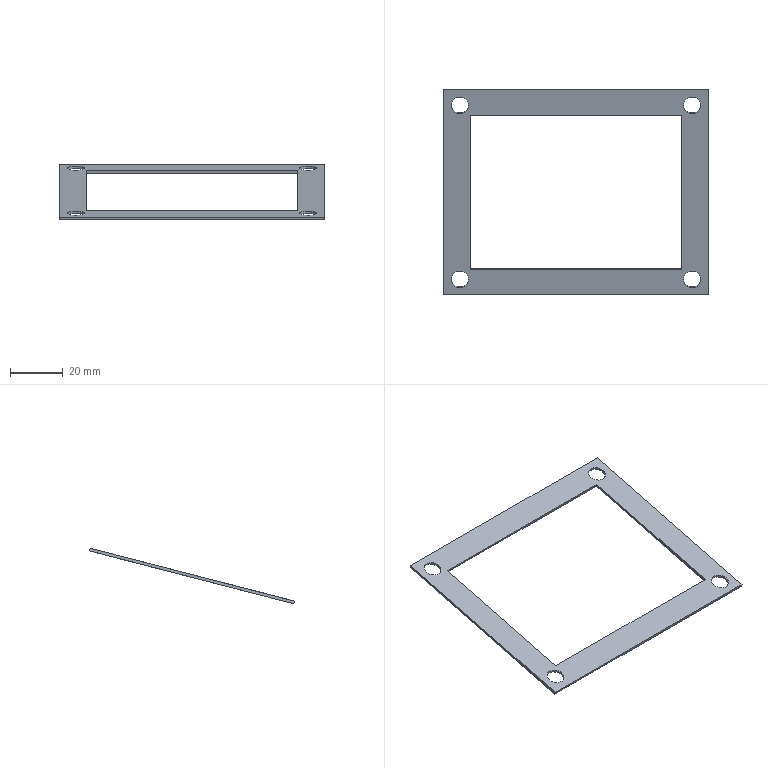Component | NX | DIANPIAN | 1 solid | 14 faces | box 100 x 77.71 x 20.97 mm | volume 3067 mm3 | plane 10 | cylinder 4 | commonest cylinder face diameters 6.5 x4
STEP:
#1=CARTESIAN_POINT('',(0.,0.,0.));
#2=DIRECTION('',(0.,0.,1.));
#3=DIRECTION('',(1.,0.,0.));
#4=AXIS2_PLACEMENT_3D('',#1,#2,#3);
#5=CARTESIAN_POINT('',(-40.,65.493,-7.056));
#6=VERTEX_POINT('',#5);
#7=CARTESIAN_POINT('',(-40.,123.588,7.944));
#8=VERTEX_POINT('',#7);
#9=CARTESIAN_POINT('',(-40.,65.493,-7.056));
#10=DIRECTION('',(0.,0.9682,0.25));
#11=VECTOR('',#10,1.);
#12=LINE('',#9,#11);
#13=CARTESIAN_POINT('',(-40.,65.243,-6.088));
#14=DIRECTION('',(-1.,0.,0.));
#15=DIRECTION('',(0.,-0.25,0.9682));
#16=AXIS2_PLACEMENT_3D('',#13,#14,#15);
#17=PLANE('',#16);
#18=CARTESIAN_POINT('',(-1.,0.));
#19=DIRECTION('',(0.,1.));
#20=VECTOR('',#19,1.);
#21=LINE('',#18,#20);
#22=(GEOMETRIC_REPRESENTATION_CONTEXT(2)PARAMETRIC_REPRESENTATION_CONTEXT()REPRESENTATION_CONTEXT('',''));
#23=DEFINITIONAL_REPRESENTATION('',(#21),#22);
#24=PCURVE('',#17,#23);
#25=CARTESIAN_POINT('',(-44.,61.62,-8.056));
#26=DIRECTION('',(0.,0.25,-0.9682));
#27=DIRECTION('',(-1.,0.,0.));
#28=AXIS2_PLACEMENT_3D('',#25,#26,#27);
#29=PLANE('',#28);
#30=CARTESIAN_POINT('',(-4.,4.));
#31=DIRECTION('',(0.,1.));
#32=VECTOR('',#31,1.);
#33=LINE('',#30,#32);
#34=(GEOMETRIC_REPRESENTATION_CONTEXT(2)PARAMETRIC_REPRESENTATION_CONTEXT()REPRESENTATION_CONTEXT('',''));
#35=DEFINITIONAL_REPRESENTATION('',(#33),#34);
#36=PCURVE('',#29,#35);
#37=SURFACE_CURVE('',#12,(#24,#36),.PCURVE_S1.);
#38=EDGE_CURVE('',#6,#8,#37,.T.);
#39=ORIENTED_EDGE('',*,*,#38,.T.);
#40=CARTESIAN_POINT('',(-40.,123.338,8.912));
#41=VERTEX_POINT('',#40);
#42=CARTESIAN_POINT('',(-40.,123.338,8.912));
#43=DIRECTION('',(0.,0.25,-0.9682));
#44=VECTOR('',#43,1.);
#45=LINE('',#42,#44);
#46=CARTESIAN_POINT('',(0.,60.));
#47=DIRECTION('',(-1.,0.));
#48=VECTOR('',#47,1.);
#49=LINE('',#46,#48);
#50=(GEOMETRIC_REPRESENTATION_CONTEXT(2)PARAMETRIC_REPRESENTATION_CONTEXT()REPRESENTATION_CONTEXT('',''));
#51=DEFINITIONAL_REPRESENTATION('',(#49),#50);
#52=PCURVE('',#17,#51);
#53=CARTESIAN_POINT('',(-40.,123.338,8.912));
#54=DIRECTION('',(0.,0.9682,0.25));
#55=DIRECTION('',(0.,-0.25,0.9682));
#56=AXIS2_PLACEMENT_3D('',#53,#54,#55);
#57=PLANE('',#56);
#58=CARTESIAN_POINT('',(0.,0.));
#59=DIRECTION('',(-1.,0.));
#60=VECTOR('',#59,1.);
#61=LINE('',#58,#60);
#62=(GEOMETRIC_REPRESENTATION_CONTEXT(2)PARAMETRIC_REPRESENTATION_CONTEXT()REPRESENTATION_CONTEXT('',''));
#63=DEFINITIONAL_REPRESENTATION('',(#61),#62);
#64=PCURVE('',#57,#63);
#65=SURFACE_CURVE('',#45,(#52,#64),.PCURVE_S1.);
#66=EDGE_CURVE('',#41,#8,#65,.T.);
#67=ORIENTED_EDGE('',*,*,#66,.F.);
#68=CARTESIAN_POINT('',(-40.,65.243,-6.088));
#69=VERTEX_POINT('',#68);
#70=CARTESIAN_POINT('',(-40.,65.243,-6.088));
#71=DIRECTION('',(0.,0.9682,0.25));
#72=VECTOR('',#71,1.);
#73=LINE('',#70,#72);
#74=CARTESIAN_POINT('',(0.,0.));
#75=DIRECTION('',(0.,1.));
#76=VECTOR('',#75,1.);
#77=LINE('',#74,#76);
#78=(GEOMETRIC_REPRESENTATION_CONTEXT(2)PARAMETRIC_REPRESENTATION_CONTEXT()REPRESENTATION_CONTEXT('',''));
#79=DEFINITIONAL_REPRESENTATION('',(#77),#78);
#80=PCURVE('',#17,#79);
#81=CARTESIAN_POINT('',(-44.,61.37,-7.088));
#82=DIRECTION('',(0.,0.25,-0.9682));
#83=DIRECTION('',(-1.,0.,0.));
#84=AXIS2_PLACEMENT_3D('',#81,#82,#83);
#85=PLANE('',#84);
#86=CARTESIAN_POINT('',(-4.,4.));
#87=DIRECTION('',(0.,1.));
#88=VECTOR('',#87,1.);
#89=LINE('',#86,#88);
#90=(GEOMETRIC_REPRESENTATION_CONTEXT(2)PARAMETRIC_REPRESENTATION_CONTEXT()REPRESENTATION_CONTEXT('',''));
#91=DEFINITIONAL_REPRESENTATION('',(#89),#90);
#92=PCURVE('',#85,#91);
#93=SURFACE_CURVE('',#73,(#80,#92),.PCURVE_S1.);
#94=EDGE_CURVE('',#69,#41,#93,.T.);
#95=ORIENTED_EDGE('',*,*,#94,.F.);
#96=CARTESIAN_POINT('',(-40.,65.243,-6.088));
#97=DIRECTION('',(0.,0.25,-0.9682));
#98=VECTOR('',#97,1.);
#99=LINE('',#96,#98);
#100=CARTESIAN_POINT('',(0.,0.));
#101=DIRECTION('',(-1.,0.));
#102=VECTOR('',#101,1.);
#103=LINE('',#100,#102);
#104=(GEOMETRIC_REPRESENTATION_CONTEXT(2)PARAMETRIC_REPRESENTATION_CONTEXT()REPRESENTATION_CONTEXT('',''));
#105=DEFINITIONAL_REPRESENTATION('',(#103),#104);
#106=PCURVE('',#17,#105);
#107=CARTESIAN_POINT('',(40.,65.243,-6.088));
#108=DIRECTION('',(0.,-0.9682,-0.25));
#109=DIRECTION('',(0.,0.25,-0.9682));
#110=AXIS2_PLACEMENT_3D('',#107,#108,#109);
#111=PLANE('',#110);
#112=CARTESIAN_POINT('',(0.,-80.));
#113=DIRECTION('',(1.,0.));
#114=VECTOR('',#113,1.);
#115=LINE('',#112,#114);
#116=(GEOMETRIC_REPRESENTATION_CONTEXT(2)PARAMETRIC_REPRESENTATION_CONTEXT()REPRESENTATION_CONTEXT('',''));
#117=DEFINITIONAL_REPRESENTATION('',(#115),#116);
#118=PCURVE('',#111,#117);
#119=SURFACE_CURVE('',#99,(#106,#118),.PCURVE_S1.);
#120=EDGE_CURVE('',#69,#6,#119,.T.);
#121=ORIENTED_EDGE('',*,*,#120,.T.);
#122=EDGE_LOOP('',(#39,#67,#95,#121));
#123=FACE_BOUND('',#122,.T.);
#124=ADVANCED_FACE('',(#123),#17,.F.);
#125=CARTESIAN_POINT('',(40.,123.588,7.944));
#126=VERTEX_POINT('',#125);
#127=CARTESIAN_POINT('',(-40.,123.588,7.944));
#128=DIRECTION('',(1.,0.,0.));
#129=VECTOR('',#128,1.);
#130=LINE('',#127,#129);
#131=CARTESIAN_POINT('',(-1.,0.));
#132=DIRECTION('',(0.,1.));
#133=VECTOR('',#132,1.);
#134=LINE('',#131,#133);
#135=(GEOMETRIC_REPRESENTATION_CONTEXT(2)PARAMETRIC_REPRESENTATION_CONTEXT()REPRESENTATION_CONTEXT('',''));
#136=DEFINITIONAL_REPRESENTATION('',(#134),#135);
#137=PCURVE('',#57,#136);
#138=CARTESIAN_POINT('',(-4.,64.));
#139=DIRECTION('',(-1.,0.));
#140=VECTOR('',#139,1.);
#141=LINE('',#138,#140);
#142=(GEOMETRIC_REPRESENTATION_CONTEXT(2)PARAMETRIC_REPRESENTATION_CONTEXT()REPRESENTATION_CONTEXT('',''));
#143=DEFINITIONAL_REPRESENTATION('',(#141),#142);
#144=PCURVE('',#29,#143);
#145=SURFACE_CURVE('',#130,(#137,#144),.PCURVE_S1.);
#146=EDGE_CURVE('',#8,#126,#145,.T.);
#147=ORIENTED_EDGE('',*,*,#146,.T.);
#148=CARTESIAN_POINT('',(40.,123.338,8.912));
#149=VERTEX_POINT('',#148);
#150=CARTESIAN_POINT('',(40.,123.338,8.912));
#151=DIRECTION('',(0.,0.25,-0.9682));
#152=VECTOR('',#151,1.);
#153=LINE('',#150,#152);
#154=CARTESIAN_POINT('',(0.,80.));
#155=DIRECTION('',(-1.,0.));
#156=VECTOR('',#155,1.);
#157=LINE('',#154,#156);
#158=(GEOMETRIC_REPRESENTATION_CONTEXT(2)PARAMETRIC_REPRESENTATION_CONTEXT()REPRESENTATION_CONTEXT('',''));
#159=DEFINITIONAL_REPRESENTATION('',(#157),#158);
#160=PCURVE('',#57,#159);
#161=CARTESIAN_POINT('',(40.,123.338,8.912));
#162=DIRECTION('',(1.,0.,0.));
#163=DIRECTION('',(0.,0.25,-0.9682));
#164=AXIS2_PLACEMENT_3D('',#161,#162,#163);
#165=PLANE('',#164);
#166=CARTESIAN_POINT('',(0.,0.));
#167=DIRECTION('',(1.,0.));
#168=VECTOR('',#167,1.);
#169=LINE('',#166,#168);
#170=(GEOMETRIC_REPRESENTATION_CONTEXT(2)PARAMETRIC_REPRESENTATION_CONTEXT()REPRESENTATION_CONTEXT('',''));
#171=DEFINITIONAL_REPRESENTATION('',(#169),#170);
#172=PCURVE('',#165,#171);
#173=SURFACE_CURVE('',#153,(#160,#172),.PCURVE_S1.);
#174=EDGE_CURVE('',#149,#126,#173,.T.);
#175=ORIENTED_EDGE('',*,*,#174,.F.);
#176=CARTESIAN_POINT('',(-40.,123.338,8.912));
#177=DIRECTION('',(1.,0.,0.));
#178=VECTOR('',#177,1.);
#179=LINE('',#176,#178);
#180=CARTESIAN_POINT('',(0.,0.));
#181=DIRECTION('',(0.,1.));
#182=VECTOR('',#181,1.);
#183=LINE('',#180,#182);
#184=(GEOMETRIC_REPRESENTATION_CONTEXT(2)PARAMETRIC_REPRESENTATION_CONTEXT()REPRESENTATION_CONTEXT('',''));
#185=DEFINITIONAL_REPRESENTATION('',(#183),#184);
#186=PCURVE('',#57,#185);
#187=CARTESIAN_POINT('',(-4.,64.));
#188=DIRECTION('',(-1.,0.));
#189=VECTOR('',#188,1.);
#190=LINE('',#187,#189);
#191=(GEOMETRIC_REPRESENTATION_CONTEXT(2)PARAMETRIC_REPRESENTATION_CONTEXT()REPRESENTATION_CONTEXT('',''));
#192=DEFINITIONAL_REPRESENTATION('',(#190),#191);
#193=PCURVE('',#85,#192);
#194=SURFACE_CURVE('',#179,(#186,#193),.PCURVE_S1.);
#195=EDGE_CURVE('',#41,#149,#194,.T.);
#196=ORIENTED_EDGE('',*,*,#195,.F.);
#197=ORIENTED_EDGE('',*,*,#66,.T.);
#198=EDGE_LOOP('',(#147,#175,#196,#197));
#199=FACE_BOUND('',#198,.T.);
#200=ADVANCED_FACE('',(#199),#57,.F.);
#201=CARTESIAN_POINT('',(40.,65.493,-7.056));
#202=VERTEX_POINT('',#201);
#203=CARTESIAN_POINT('',(40.,123.588,7.944));
#204=DIRECTION('',(0.,-0.9682,-0.25));
#205=VECTOR('',#204,1.);
#206=LINE('',#203,#205);
#207=CARTESIAN_POINT('',(1.,0.));
#208=DIRECTION('',(0.,-1.));
#209=VECTOR('',#208,1.);
#210=LINE('',#207,#209);
#211=(GEOMETRIC_REPRESENTATION_CONTEXT(2)PARAMETRIC_REPRESENTATION_CONTEXT()REPRESENTATION_CONTEXT('',''));
#212=DEFINITIONAL_REPRESENTATION('',(#210),#211);
#213=PCURVE('',#165,#212);
#214=CARTESIAN_POINT('',(-84.,64.));
#215=DIRECTION('',(0.,-1.));
#216=VECTOR('',#215,1.);
#217=LINE('',#214,#216);
#218=(GEOMETRIC_REPRESENTATION_CONTEXT(2)PARAMETRIC_REPRESENTATION_CONTEXT()REPRESENTATION_CONTEXT('',''));
#219=DEFINITIONAL_REPRESENTATION('',(#217),#218);
#220=PCURVE('',#29,#219);
#221=SURFACE_CURVE('',#206,(#213,#220),.PCURVE_S1.);
#222=EDGE_CURVE('',#126,#202,#221,.T.);
#223=ORIENTED_EDGE('',*,*,#222,.T.);
#224=CARTESIAN_POINT('',(40.,65.243,-6.088));
#225=VERTEX_POINT('',#224);
#226=CARTESIAN_POINT('',(40.,65.243,-6.088));
#227=DIRECTION('',(0.,0.25,-0.9682));
#228=VECTOR('',#227,1.);
#229=LINE('',#226,#228);
#230=CARTESIAN_POINT('',(0.,-60.));
#231=DIRECTION('',(1.,0.));
#232=VECTOR('',#231,1.);
#233=LINE('',#230,#232);
#234=(GEOMETRIC_REPRESENTATION_CONTEXT(2)PARAMETRIC_REPRESENTATION_CONTEXT()REPRESENTATION_CONTEXT('',''));
#235=DEFINITIONAL_REPRESENTATION('',(#233),#234);
#236=PCURVE('',#165,#235);
#237=CARTESIAN_POINT('',(0.,0.));
#238=DIRECTION('',(1.,0.));
#239=VECTOR('',#238,1.);
#240=LINE('',#237,#239);
#241=(GEOMETRIC_REPRESENTATION_CONTEXT(2)PARAMETRIC_REPRESENTATION_CONTEXT()REPRESENTATION_CONTEXT('',''));
#242=DEFINITIONAL_REPRESENTATION('',(#240),#241);
#243=PCURVE('',#111,#242);
#244=SURFACE_CURVE('',#229,(#236,#243),.PCURVE_S1.);
#245=EDGE_CURVE('',#225,#202,#244,.T.);
#246=ORIENTED_EDGE('',*,*,#245,.F.);
#247=CARTESIAN_POINT('',(40.,123.338,8.912));
#248=DIRECTION('',(0.,-0.9682,-0.25));
#249=VECTOR('',#248,1.);
#250=LINE('',#247,#249);
#251=CARTESIAN_POINT('',(0.,0.));
#252=DIRECTION('',(0.,-1.));
#253=VECTOR('',#252,1.);
#254=LINE('',#251,#253);
#255=(GEOMETRIC_REPRESENTATION_CONTEXT(2)PARAMETRIC_REPRESENTATION_CONTEXT()REPRESENTATION_CONTEXT('',''));
#256=DEFINITIONAL_REPRESENTATION('',(#254),#255);
#257=PCURVE('',#165,#256);
#258=CARTESIAN_POINT('',(-84.,64.));
#259=DIRECTION('',(0.,-1.));
#260=VECTOR('',#259,1.);
#261=LINE('',#258,#260);
#262=(GEOMETRIC_REPRESENTATION_CONTEXT(2)PARAMETRIC_REPRESENTATION_CONTEXT()REPRESENTATION_CONTEXT('',''));
#263=DEFINITIONAL_REPRESENTATION('',(#261),#262);
#264=PCURVE('',#85,#263);
#265=SURFACE_CURVE('',#250,(#257,#264),.PCURVE_S1.);
#266=EDGE_CURVE('',#149,#225,#265,.T.);
#267=ORIENTED_EDGE('',*,*,#266,.F.);
#268=ORIENTED_EDGE('',*,*,#174,.T.);
#269=EDGE_LOOP('',(#223,#246,#267,#268));
#270=FACE_BOUND('',#269,.T.);
#271=ADVANCED_FACE('',(#270),#165,.F.);
#272=CARTESIAN_POINT('',(-50.,133.27,10.444));
#273=VERTEX_POINT('',#272);
#274=CARTESIAN_POINT('',(-50.,55.81,-9.556));
#275=VERTEX_POINT('',#274);
#276=CARTESIAN_POINT('',(-50.,133.27,10.444));
#277=DIRECTION('',(0.,-0.9682,-0.25));
#278=VECTOR('',#277,1.);
#279=LINE('',#276,#278);
#280=CARTESIAN_POINT('',(-50.,133.02,11.412));
#281=DIRECTION('',(1.,0.,0.));
#282=DIRECTION('',(0.,0.25,-0.9682));
#283=AXIS2_PLACEMENT_3D('',#280,#281,#282);
#284=PLANE('',#283);
#285=CARTESIAN_POINT('',(1.,-0.));
#286=DIRECTION('',(0.,-1.));
#287=VECTOR('',#286,1.);
#288=LINE('',#285,#287);
#289=(GEOMETRIC_REPRESENTATION_CONTEXT(2)PARAMETRIC_REPRESENTATION_CONTEXT()REPRESENTATION_CONTEXT('',''));
#290=DEFINITIONAL_REPRESENTATION('',(#288),#289);
#291=PCURVE('',#284,#290);
#292=CARTESIAN_POINT('',(6.,74.));
#293=DIRECTION('',(0.,-1.));
#294=VECTOR('',#293,1.);
#295=LINE('',#292,#294);
#296=(GEOMETRIC_REPRESENTATION_CONTEXT(2)PARAMETRIC_REPRESENTATION_CONTEXT()REPRESENTATION_CONTEXT('',''));
#297=DEFINITIONAL_REPRESENTATION('',(#295),#296);
#298=PCURVE('',#29,#297);
#299=SURFACE_CURVE('',#279,(#291,#298),.PCURVE_S1.);
#300=EDGE_CURVE('',#273,#275,#299,.T.);
#301=ORIENTED_EDGE('',*,*,#300,.T.);
#302=CARTESIAN_POINT('',(-50.,55.56,-8.588));
#303=VERTEX_POINT('',#302);
#304=CARTESIAN_POINT('',(-50.,55.56,-8.588));
#305=DIRECTION('',(0.,0.25,-0.9682));
#306=VECTOR('',#305,1.);
#307=LINE('',#304,#306);
#308=CARTESIAN_POINT('',(-0.,-80.));
#309=DIRECTION('',(1.,0.));
#310=VECTOR('',#309,1.);
#311=LINE('',#308,#310);
#312=(GEOMETRIC_REPRESENTATION_CONTEXT(2)PARAMETRIC_REPRESENTATION_CONTEXT()REPRESENTATION_CONTEXT('',''));
#313=DEFINITIONAL_REPRESENTATION('',(#311),#312);
#314=PCURVE('',#284,#313);
#315=CARTESIAN_POINT('',(-50.,55.56,-8.588));
#316=DIRECTION('',(0.,0.9682,0.25));
#317=DIRECTION('',(0.,-0.25,0.9682));
#318=AXIS2_PLACEMENT_3D('',#315,#316,#317);
#319=PLANE('',#318);
#320=CARTESIAN_POINT('',(0.,0.));
#321=DIRECTION('',(-1.,0.));
#322=VECTOR('',#321,1.);
#323=LINE('',#320,#322);
#324=(GEOMETRIC_REPRESENTATION_CONTEXT(2)PARAMETRIC_REPRESENTATION_CONTEXT()REPRESENTATION_CONTEXT('',''));
#325=DEFINITIONAL_REPRESENTATION('',(#323),#324);
#326=PCURVE('',#319,#325);
#327=SURFACE_CURVE('',#307,(#314,#326),.PCURVE_S1.);
#328=EDGE_CURVE('',#303,#275,#327,.T.);
#329=ORIENTED_EDGE('',*,*,#328,.F.);
#330=CARTESIAN_POINT('',(-50.,133.02,11.412));
#331=VERTEX_POINT('',#330);
#332=CARTESIAN_POINT('',(-50.,133.02,11.412));
#333=DIRECTION('',(0.,-0.9682,-0.25));
#334=VECTOR('',#333,1.);
#335=LINE('',#332,#334);
#336=CARTESIAN_POINT('',(0.,0.));
#337=DIRECTION('',(0.,-1.));
#338=VECTOR('',#337,1.);
#339=LINE('',#336,#338);
#340=(GEOMETRIC_REPRESENTATION_CONTEXT(2)PARAMETRIC_REPRESENTATION_CONTEXT()REPRESENTATION_CONTEXT('',''));
#341=DEFINITIONAL_REPRESENTATION('',(#339),#340);
#342=PCURVE('',#284,#341);
#343=CARTESIAN_POINT('',(6.,74.));
#344=DIRECTION('',(0.,-1.));
#345=VECTOR('',#344,1.);
#346=LINE('',#343,#345);
#347=(GEOMETRIC_REPRESENTATION_CONTEXT(2)PARAMETRIC_REPRESENTATION_CONTEXT()REPRESENTATION_CONTEXT('',''));
#348=DEFINITIONAL_REPRESENTATION('',(#346),#347);
#349=PCURVE('',#85,#348);
#350=SURFACE_CURVE('',#335,(#342,#349),.PCURVE_S1.);
#351=EDGE_CURVE('',#331,#303,#350,.T.);
#352=ORIENTED_EDGE('',*,*,#351,.F.);
#353=CARTESIAN_POINT('',(-50.,133.02,11.412));
#354=DIRECTION('',(0.,0.25,-0.9682));
#355=VECTOR('',#354,1.);
#356=LINE('',#353,#355);
#357=CARTESIAN_POINT('',(0.,0.));
#358=DIRECTION('',(1.,0.));
#359=VECTOR('',#358,1.);
#360=LINE('',#357,#359);
#361=(GEOMETRIC_REPRESENTATION_CONTEXT(2)PARAMETRIC_REPRESENTATION_CONTEXT()REPRESENTATION_CONTEXT('',''));
#362=DEFINITIONAL_REPRESENTATION('',(#360),#361);
#363=PCURVE('',#284,#362);
#364=CARTESIAN_POINT('',(50.,133.02,11.412));
#365=DIRECTION('',(0.,-0.9682,-0.25));
#366=DIRECTION('',(0.,0.25,-0.9682));
#367=AXIS2_PLACEMENT_3D('',#364,#365,#366);
#368=PLANE('',#367);
#369=CARTESIAN_POINT('',(0.,-100.));
#370=DIRECTION('',(1.,0.));
#371=VECTOR('',#370,1.);
#372=LINE('',#369,#371);
#373=(GEOMETRIC_REPRESENTATION_CONTEXT(2)PARAMETRIC_REPRESENTATION_CONTEXT()REPRESENTATION_CONTEXT('',''));
#374=DEFINITIONAL_REPRESENTATION('',(#372),#373);
#375=PCURVE('',#368,#374);
#376=SURFACE_CURVE('',#356,(#363,#375),.PCURVE_S1.);
#377=EDGE_CURVE('',#331,#273,#376,.T.);
#378=ORIENTED_EDGE('',*,*,#377,.T.);
#379=EDGE_LOOP('',(#301,#329,#352,#378));
#380=FACE_BOUND('',#379,.T.);
#381=ADVANCED_FACE('',(#380),#284,.F.);
#382=CARTESIAN_POINT('',(50.,55.81,-9.556));
#383=VERTEX_POINT('',#382);
#384=CARTESIAN_POINT('',(-50.,55.81,-9.556));
#385=DIRECTION('',(1.,0.,0.));
#386=VECTOR('',#385,1.);
#387=LINE('',#384,#386);
#388=CARTESIAN_POINT('',(-1.,0.));
#389=DIRECTION('',(0.,1.));
#390=VECTOR('',#389,1.);
#391=LINE('',#388,#390);
#392=(GEOMETRIC_REPRESENTATION_CONTEXT(2)PARAMETRIC_REPRESENTATION_CONTEXT()REPRESENTATION_CONTEXT('',''));
#393=DEFINITIONAL_REPRESENTATION('',(#391),#392);
#394=PCURVE('',#319,#393);
#395=CARTESIAN_POINT('',(6.,-6.));
#396=DIRECTION('',(-1.,0.));
#397=VECTOR('',#396,1.);
#398=LINE('',#395,#397);
#399=(GEOMETRIC_REPRESENTATION_CONTEXT(2)PARAMETRIC_REPRESENTATION_CONTEXT()REPRESENTATION_CONTEXT('',''));
#400=DEFINITIONAL_REPRESENTATION('',(#398),#399);
#401=PCURVE('',#29,#400);
#402=SURFACE_CURVE('',#387,(#394,#401),.PCURVE_S1.);
#403=EDGE_CURVE('',#275,#383,#402,.T.);
#404=ORIENTED_EDGE('',*,*,#403,.T.);
#405=CARTESIAN_POINT('',(50.,55.56,-8.588));
#406=VERTEX_POINT('',#405);
#407=CARTESIAN_POINT('',(50.,55.56,-8.588));
#408=DIRECTION('',(0.,0.25,-0.9682));
#409=VECTOR('',#408,1.);
#410=LINE('',#407,#409);
#411=CARTESIAN_POINT('',(0.,100.));
#412=DIRECTION('',(-1.,0.));
#413=VECTOR('',#412,1.);
#414=LINE('',#411,#413);
#415=(GEOMETRIC_REPRESENTATION_CONTEXT(2)PARAMETRIC_REPRESENTATION_CONTEXT()REPRESENTATION_CONTEXT('',''));
#416=DEFINITIONAL_REPRESENTATION('',(#414),#415);
#417=PCURVE('',#319,#416);
#418=CARTESIAN_POINT('',(50.,55.56,-8.588));
#419=DIRECTION('',(-1.,0.,0.));
#420=DIRECTION('',(0.,-0.25,0.9682));
#421=AXIS2_PLACEMENT_3D('',#418,#419,#420);
#422=PLANE('',#421);
#423=CARTESIAN_POINT('',(0.,0.));
#424=DIRECTION('',(-1.,0.));
#425=VECTOR('',#424,1.);
#426=LINE('',#423,#425);
#427=(GEOMETRIC_REPRESENTATION_CONTEXT(2)PARAMETRIC_REPRESENTATION_CONTEXT()REPRESENTATION_CONTEXT('',''));
#428=DEFINITIONAL_REPRESENTATION('',(#426),#427);
#429=PCURVE('',#422,#428);
#430=SURFACE_CURVE('',#410,(#417,#429),.PCURVE_S1.);
#431=EDGE_CURVE('',#406,#383,#430,.T.);
#432=ORIENTED_EDGE('',*,*,#431,.F.);
#433=CARTESIAN_POINT('',(-50.,55.56,-8.588));
#434=DIRECTION('',(1.,0.,0.));
#435=VECTOR('',#434,1.);
#436=LINE('',#433,#435);
#437=CARTESIAN_POINT('',(0.,0.));
#438=DIRECTION('',(0.,1.));
#439=VECTOR('',#438,1.);
#440=LINE('',#437,#439);
#441=(GEOMETRIC_REPRESENTATION_CONTEXT(2)PARAMETRIC_REPRESENTATION_CONTEXT()REPRESENTATION_CONTEXT('',''));
#442=DEFINITIONAL_REPRESENTATION('',(#440),#441);
#443=PCURVE('',#319,#442);
#444=CARTESIAN_POINT('',(6.,-6.));
#445=DIRECTION('',(-1.,0.));
#446=VECTOR('',#445,1.);
#447=LINE('',#444,#446);
#448=(GEOMETRIC_REPRESENTATION_CONTEXT(2)PARAMETRIC_REPRESENTATION_CONTEXT()REPRESENTATION_CONTEXT('',''));
#449=DEFINITIONAL_REPRESENTATION('',(#447),#448);
#450=PCURVE('',#85,#449);
#451=SURFACE_CURVE('',#436,(#443,#450),.PCURVE_S1.);
#452=EDGE_CURVE('',#303,#406,#451,.T.);
#453=ORIENTED_EDGE('',*,*,#452,.F.);
#454=ORIENTED_EDGE('',*,*,#328,.T.);
#455=EDGE_LOOP('',(#404,#432,#453,#454));
#456=FACE_BOUND('',#455,.T.);
#457=ADVANCED_FACE('',(#456),#319,.F.);
#458=CARTESIAN_POINT('',(50.,133.27,10.444));
#459=VERTEX_POINT('',#458);
#460=CARTESIAN_POINT('',(50.,55.81,-9.556));
#461=DIRECTION('',(0.,0.9682,0.25));
#462=VECTOR('',#461,1.);
#463=LINE('',#460,#462);
#464=CARTESIAN_POINT('',(-1.,0.));
#465=DIRECTION('',(0.,1.));
#466=VECTOR('',#465,1.);
#467=LINE('',#464,#466);
#468=(GEOMETRIC_REPRESENTATION_CONTEXT(2)PARAMETRIC_REPRESENTATION_CONTEXT()REPRESENTATION_CONTEXT('',''));
#469=DEFINITIONAL_REPRESENTATION('',(#467),#468);
#470=PCURVE('',#422,#469);
#471=CARTESIAN_POINT('',(-94.,-6.));
#472=DIRECTION('',(0.,1.));
#473=VECTOR('',#472,1.);
#474=LINE('',#471,#473);
#475=(GEOMETRIC_REPRESENTATION_CONTEXT(2)PARAMETRIC_REPRESENTATION_CONTEXT()REPRESENTATION_CONTEXT('',''));
#476=DEFINITIONAL_REPRESENTATION('',(#474),#475);
#477=PCURVE('',#29,#476);
#478=SURFACE_CURVE('',#463,(#470,#477),.PCURVE_S1.);
#479=EDGE_CURVE('',#383,#459,#478,.T.);
#480=ORIENTED_EDGE('',*,*,#479,.T.);
#481=CARTESIAN_POINT('',(50.,133.02,11.412));
#482=VERTEX_POINT('',#481);
#483=CARTESIAN_POINT('',(50.,133.02,11.412));
#484=DIRECTION('',(0.,0.25,-0.9682));
#485=VECTOR('',#484,1.);
#486=LINE('',#483,#485);
#487=CARTESIAN_POINT('',(-0.,80.));
#488=DIRECTION('',(-1.,0.));
#489=VECTOR('',#488,1.);
#490=LINE('',#487,#489);
#491=(GEOMETRIC_REPRESENTATION_CONTEXT(2)PARAMETRIC_REPRESENTATION_CONTEXT()REPRESENTATION_CONTEXT('',''));
#492=DEFINITIONAL_REPRESENTATION('',(#490),#491);
#493=PCURVE('',#422,#492);
#494=CARTESIAN_POINT('',(0.,0.));
#495=DIRECTION('',(1.,0.));
#496=VECTOR('',#495,1.);
#497=LINE('',#494,#496);
#498=(GEOMETRIC_REPRESENTATION_CONTEXT(2)PARAMETRIC_REPRESENTATION_CONTEXT()REPRESENTATION_CONTEXT('',''));
#499=DEFINITIONAL_REPRESENTATION('',(#497),#498);
#500=PCURVE('',#368,#499);
#501=SURFACE_CURVE('',#486,(#493,#500),.PCURVE_S1.);
#502=EDGE_CURVE('',#482,#459,#501,.T.);
#503=ORIENTED_EDGE('',*,*,#502,.F.);
#504=CARTESIAN_POINT('',(50.,55.56,-8.588));
#505=DIRECTION('',(0.,0.9682,0.25));
#506=VECTOR('',#505,1.);
#507=LINE('',#504,#506);
#508=CARTESIAN_POINT('',(0.,0.));
#509=DIRECTION('',(0.,1.));
#510=VECTOR('',#509,1.);
#511=LINE('',#508,#510);
#512=(GEOMETRIC_REPRESENTATION_CONTEXT(2)PARAMETRIC_REPRESENTATION_CONTEXT()REPRESENTATION_CONTEXT('',''));
#513=DEFINITIONAL_REPRESENTATION('',(#511),#512);
#514=PCURVE('',#422,#513);
#515=CARTESIAN_POINT('',(-94.,-6.));
#516=DIRECTION('',(0.,1.));
#517=VECTOR('',#516,1.);
#518=LINE('',#515,#517);
#519=(GEOMETRIC_REPRESENTATION_CONTEXT(2)PARAMETRIC_REPRESENTATION_CONTEXT()REPRESENTATION_CONTEXT('',''));
#520=DEFINITIONAL_REPRESENTATION('',(#518),#519);
#521=PCURVE('',#85,#520);
#522=SURFACE_CURVE('',#507,(#514,#521),.PCURVE_S1.);
#523=EDGE_CURVE('',#406,#482,#522,.T.);
#524=ORIENTED_EDGE('',*,*,#523,.F.);
#525=ORIENTED_EDGE('',*,*,#431,.T.);
#526=EDGE_LOOP('',(#480,#503,#524,#525));
#527=FACE_BOUND('',#526,.T.);
#528=ADVANCED_FACE('',(#527),#422,.F.);
#529=CARTESIAN_POINT('',(40.75,127.211,9.912));
#530=VERTEX_POINT('',#529);
#531=CARTESIAN_POINT('',(44.,127.211,9.912));
#532=DIRECTION('',(0.,0.25,-0.9682));
#533=DIRECTION('',(-1.,0.,0.));
#534=AXIS2_PLACEMENT_3D('',#531,#532,#533);
#535=CIRCLE('',#534,3.25);
#536=CARTESIAN_POINT('',(44.,127.211,9.912));
#537=DIRECTION('',(0.,0.25,-0.9682));
#538=DIRECTION('',(-1.,0.,0.));
#539=AXIS2_PLACEMENT_3D('',#536,#537,#538);
#540=CYLINDRICAL_SURFACE('',#539,3.25);
#541=CARTESIAN_POINT('',(0.,0.));
#542=DIRECTION('',(1.,0.));
#543=VECTOR('',#542,1.);
#544=LINE('',#541,#543);
#545=(GEOMETRIC_REPRESENTATION_CONTEXT(2)PARAMETRIC_REPRESENTATION_CONTEXT()REPRESENTATION_CONTEXT('',''));
#546=DEFINITIONAL_REPRESENTATION('',(#544),#545);
#547=PCURVE('',#540,#546);
#548=CARTESIAN_POINT('',(-88.,68.));
#549=DIRECTION('',(1.,0.));
#550=AXIS2_PLACEMENT_2D('',#548,#549);
#551=CIRCLE('',#550,3.25);
#552=(GEOMETRIC_REPRESENTATION_CONTEXT(2)PARAMETRIC_REPRESENTATION_CONTEXT()REPRESENTATION_CONTEXT('',''));
#553=DEFINITIONAL_REPRESENTATION('',(#551),#552);
#554=PCURVE('',#85,#553);
#555=SURFACE_CURVE('',#535,(#547,#554),.PCURVE_S1.);
#556=EDGE_CURVE('',#530,#530,#555,.T.);
#557=ORIENTED_EDGE('',*,*,#556,.T.);
#558=CARTESIAN_POINT('',(40.75,127.461,8.944));
#559=VERTEX_POINT('',#558);
#560=CARTESIAN_POINT('',(40.75,127.211,9.912));
#561=CARTESIAN_POINT('',(40.75,127.461,8.944));
#562=B_SPLINE_CURVE_WITH_KNOTS('',1,(#560,#561),.UNSPECIFIED.,.F.,.F.,(2,2),(0.,1.),.PIECEWISE_BEZIER_KNOTS.);
#563=CARTESIAN_POINT('',(6.283,0.));
#564=DIRECTION('',(0.,1.));
#565=VECTOR('',#564,1.);
#566=LINE('',#563,#565);
#567=(GEOMETRIC_REPRESENTATION_CONTEXT(2)PARAMETRIC_REPRESENTATION_CONTEXT()REPRESENTATION_CONTEXT('',''));
#568=DEFINITIONAL_REPRESENTATION('',(#566),#567);
#569=PCURVE('',#540,#568);
#570=CARTESIAN_POINT('',(0.,0.));
#571=DIRECTION('',(0.,1.));
#572=VECTOR('',#571,1.);
#573=LINE('',#570,#572);
#574=(GEOMETRIC_REPRESENTATION_CONTEXT(2)PARAMETRIC_REPRESENTATION_CONTEXT()REPRESENTATION_CONTEXT('',''));
#575=DEFINITIONAL_REPRESENTATION('',(#573),#574);
#576=PCURVE('',#540,#575);
#577=SEAM_CURVE('',#562,(#569,#576),.PCURVE_S1.);
#578=EDGE_CURVE('',#530,#559,#577,.T.);
#579=ORIENTED_EDGE('',*,*,#578,.T.);
#580=CARTESIAN_POINT('',(44.,127.461,8.944));
#581=DIRECTION('',(0.,0.25,-0.9682));
#582=DIRECTION('',(-1.,0.,0.));
#583=AXIS2_PLACEMENT_3D('',#580,#581,#582);
#584=CIRCLE('',#583,3.25);
#585=CARTESIAN_POINT('',(0.,1.));
#586=DIRECTION('',(1.,0.));
#587=VECTOR('',#586,1.);
#588=LINE('',#585,#587);
#589=(GEOMETRIC_REPRESENTATION_CONTEXT(2)PARAMETRIC_REPRESENTATION_CONTEXT()REPRESENTATION_CONTEXT('',''));
#590=DEFINITIONAL_REPRESENTATION('',(#588),#589);
#591=PCURVE('',#540,#590);
#592=CARTESIAN_POINT('',(-88.,68.));
#593=DIRECTION('',(1.,0.));
#594=AXIS2_PLACEMENT_2D('',#592,#593);
#595=CIRCLE('',#594,3.25);
#596=(GEOMETRIC_REPRESENTATION_CONTEXT(2)PARAMETRIC_REPRESENTATION_CONTEXT()REPRESENTATION_CONTEXT('',''));
#597=DEFINITIONAL_REPRESENTATION('',(#595),#596);
#598=PCURVE('',#29,#597);
#599=SURFACE_CURVE('',#584,(#591,#598),.PCURVE_S1.);
#600=EDGE_CURVE('',#559,#559,#599,.T.);
#601=ORIENTED_EDGE('',*,*,#600,.F.);
#602=ORIENTED_EDGE('',*,*,#578,.F.);
#603=EDGE_LOOP('',(#557,#579,#601,#602));
#604=FACE_BOUND('',#603,.F.);
#605=ADVANCED_FACE('',(#604),#540,.F.);
#606=CARTESIAN_POINT('',(40.75,61.37,-7.088));
#607=VERTEX_POINT('',#606);
#608=CARTESIAN_POINT('',(44.,61.37,-7.088));
#609=DIRECTION('',(0.,-0.25,0.9682));
#610=DIRECTION('',(-1.,0.,0.));
#611=AXIS2_PLACEMENT_3D('',#608,#609,#610);
#612=CIRCLE('',#611,3.25);
#613=CARTESIAN_POINT('',(44.,61.37,-7.088));
#614=DIRECTION('',(0.,0.25,-0.9682));
#615=DIRECTION('',(-1.,0.,0.));
#616=AXIS2_PLACEMENT_3D('',#613,#614,#615);
#617=CYLINDRICAL_SURFACE('',#616,3.25);
#618=CARTESIAN_POINT('',(6.283,0.));
#619=DIRECTION('',(-1.,0.));
#620=VECTOR('',#619,1.);
#621=LINE('',#618,#620);
#622=(GEOMETRIC_REPRESENTATION_CONTEXT(2)PARAMETRIC_REPRESENTATION_CONTEXT()REPRESENTATION_CONTEXT('',''));
#623=DEFINITIONAL_REPRESENTATION('',(#621),#622);
#624=PCURVE('',#617,#623);
#625=CARTESIAN_POINT('',(-84.75,0.));
#626=CARTESIAN_POINT('',(-84.75,-5.629));
#627=CARTESIAN_POINT('',(-89.625,-2.815));
#628=CARTESIAN_POINT('',(-94.5,-0.));
#629=CARTESIAN_POINT('',(-89.625,2.815));
#630=CARTESIAN_POINT('',(-84.75,5.629));
#631=CARTESIAN_POINT('',(-84.75,0.));
#632=(BOUNDED_CURVE()B_SPLINE_CURVE(2,(#625,#626,#627,#628,#629,#630,#631),.UNSPECIFIED.,.T.,.F.)B_SPLINE_CURVE_WITH_KNOTS((1,2,2,2,2,1),(-2.094,0.,2.094,4.189,6.283,8.378),.UNSPECIFIED.)CURVE()GEOMETRIC_REPRESENTATION_ITEM()RATIONAL_B_SPLINE_CURVE((1.,0.5,1.,0.5,1.,0.5,1.))REPRESENTATION_ITEM(''));
#633=(GEOMETRIC_REPRESENTATION_CONTEXT(2)PARAMETRIC_REPRESENTATION_CONTEXT()REPRESENTATION_CONTEXT('',''));
#634=DEFINITIONAL_REPRESENTATION('',(#632),#633);
#635=PCURVE('',#85,#634);
#636=SURFACE_CURVE('',#612,(#624,#635),.PCURVE_S1.);
#637=EDGE_CURVE('',#607,#607,#636,.T.);
#638=ORIENTED_EDGE('',*,*,#637,.F.);
#639=CARTESIAN_POINT('',(40.75,61.62,-8.056));
#640=VERTEX_POINT('',#639);
#641=CARTESIAN_POINT('',(40.75,61.37,-7.088));
#642=CARTESIAN_POINT('',(40.75,61.62,-8.056));
#643=B_SPLINE_CURVE_WITH_KNOTS('',1,(#641,#642),.UNSPECIFIED.,.F.,.F.,(2,2),(0.,1.),.PIECEWISE_BEZIER_KNOTS.);
#644=CARTESIAN_POINT('',(6.283,0.));
#645=DIRECTION('',(0.,1.));
#646=VECTOR('',#645,1.);
#647=LINE('',#644,#646);
#648=(GEOMETRIC_REPRESENTATION_CONTEXT(2)PARAMETRIC_REPRESENTATION_CONTEXT()REPRESENTATION_CONTEXT('',''));
#649=DEFINITIONAL_REPRESENTATION('',(#647),#648);
#650=PCURVE('',#617,#649);
#651=CARTESIAN_POINT('',(0.,0.));
#652=DIRECTION('',(0.,1.));
#653=VECTOR('',#652,1.);
#654=LINE('',#651,#653);
#655=(GEOMETRIC_REPRESENTATION_CONTEXT(2)PARAMETRIC_REPRESENTATION_CONTEXT()REPRESENTATION_CONTEXT('',''));
#656=DEFINITIONAL_REPRESENTATION('',(#654),#655);
#657=PCURVE('',#617,#656);
#658=SEAM_CURVE('',#643,(#650,#657),.PCURVE_S1.);
#659=EDGE_CURVE('',#607,#640,#658,.T.);
#660=ORIENTED_EDGE('',*,*,#659,.T.);
#661=CARTESIAN_POINT('',(44.,61.62,-8.056));
#662=DIRECTION('',(0.,-0.25,0.9682));
#663=DIRECTION('',(-1.,0.,0.));
#664=AXIS2_PLACEMENT_3D('',#661,#662,#663);
#665=CIRCLE('',#664,3.25);
#666=CARTESIAN_POINT('',(6.283,1.));
#667=DIRECTION('',(-1.,0.));
#668=VECTOR('',#667,1.);
#669=LINE('',#666,#668);
#670=(GEOMETRIC_REPRESENTATION_CONTEXT(2)PARAMETRIC_REPRESENTATION_CONTEXT()REPRESENTATION_CONTEXT('',''));
#671=DEFINITIONAL_REPRESENTATION('',(#669),#670);
#672=PCURVE('',#617,#671);
#673=CARTESIAN_POINT('',(-84.75,0.));
#674=CARTESIAN_POINT('',(-84.75,-5.629));
#675=CARTESIAN_POINT('',(-89.625,-2.815));
#676=CARTESIAN_POINT('',(-94.5,-0.));
#677=CARTESIAN_POINT('',(-89.625,2.815));
#678=CARTESIAN_POINT('',(-84.75,5.629));
#679=CARTESIAN_POINT('',(-84.75,0.));
#680=(BOUNDED_CURVE()B_SPLINE_CURVE(2,(#673,#674,#675,#676,#677,#678,#679),.UNSPECIFIED.,.T.,.F.)B_SPLINE_CURVE_WITH_KNOTS((1,2,2,2,2,1),(-2.094,0.,2.094,4.189,6.283,8.378),.UNSPECIFIED.)CURVE()GEOMETRIC_REPRESENTATION_ITEM()RATIONAL_B_SPLINE_CURVE((1.,0.5,1.,0.5,1.,0.5,1.))REPRESENTATION_ITEM(''));
#681=(GEOMETRIC_REPRESENTATION_CONTEXT(2)PARAMETRIC_REPRESENTATION_CONTEXT()REPRESENTATION_CONTEXT('',''));
#682=DEFINITIONAL_REPRESENTATION('',(#680),#681);
#683=PCURVE('',#29,#682);
#684=SURFACE_CURVE('',#665,(#672,#683),.PCURVE_S1.);
#685=EDGE_CURVE('',#640,#640,#684,.T.);
#686=ORIENTED_EDGE('',*,*,#685,.T.);
#687=ORIENTED_EDGE('',*,*,#659,.F.);
#688=EDGE_LOOP('',(#638,#660,#686,#687));
#689=FACE_BOUND('',#688,.F.);
#690=ADVANCED_FACE('',(#689),#617,.F.);
#691=CARTESIAN_POINT('',(-40.75,127.211,9.912));
#692=VERTEX_POINT('',#691);
#693=CARTESIAN_POINT('',(-44.,127.211,9.912));
#694=DIRECTION('',(0.,-0.25,0.9682));
#695=DIRECTION('',(1.,0.,0.));
#696=AXIS2_PLACEMENT_3D('',#693,#694,#695);
#697=CIRCLE('',#696,3.25);
#698=CARTESIAN_POINT('',(-44.,127.211,9.912));
#699=DIRECTION('',(0.,0.25,-0.9682));
#700=DIRECTION('',(-1.,0.,0.));
#701=AXIS2_PLACEMENT_3D('',#698,#699,#700);
#702=CYLINDRICAL_SURFACE('',#701,3.25);
#703=CARTESIAN_POINT('',(9.425,0.));
#704=DIRECTION('',(-1.,0.));
#705=VECTOR('',#704,1.);
#706=LINE('',#703,#705);
#707=(GEOMETRIC_REPRESENTATION_CONTEXT(2)PARAMETRIC_REPRESENTATION_CONTEXT()REPRESENTATION_CONTEXT('',''));
#708=DEFINITIONAL_REPRESENTATION('',(#706),#707);
#709=PCURVE('',#702,#708);
#710=CARTESIAN_POINT('',(-3.25,68.));
#711=CARTESIAN_POINT('',(-3.25,73.629));
#712=CARTESIAN_POINT('',(1.625,70.815));
#713=CARTESIAN_POINT('',(6.5,68.));
#714=CARTESIAN_POINT('',(1.625,65.185));
#715=CARTESIAN_POINT('',(-3.25,62.371));
#716=CARTESIAN_POINT('',(-3.25,68.));
#717=(BOUNDED_CURVE()B_SPLINE_CURVE(2,(#710,#711,#712,#713,#714,#715,#716),.UNSPECIFIED.,.T.,.F.)B_SPLINE_CURVE_WITH_KNOTS((1,2,2,2,2,1),(-2.094,0.,2.094,4.189,6.283,8.378),.UNSPECIFIED.)CURVE()GEOMETRIC_REPRESENTATION_ITEM()RATIONAL_B_SPLINE_CURVE((1.,0.5,1.,0.5,1.,0.5,1.))REPRESENTATION_ITEM(''));
#718=(GEOMETRIC_REPRESENTATION_CONTEXT(2)PARAMETRIC_REPRESENTATION_CONTEXT()REPRESENTATION_CONTEXT('',''));
#719=DEFINITIONAL_REPRESENTATION('',(#717),#718);
#720=PCURVE('',#85,#719);
#721=SURFACE_CURVE('',#697,(#709,#720),.PCURVE_S1.);
#722=EDGE_CURVE('',#692,#692,#721,.T.);
#723=ORIENTED_EDGE('',*,*,#722,.F.);
#724=CARTESIAN_POINT('',(-40.75,127.461,8.944));
#725=VERTEX_POINT('',#724);
#726=CARTESIAN_POINT('',(-40.75,127.211,9.912));
#727=CARTESIAN_POINT('',(-40.75,127.461,8.944));
#728=B_SPLINE_CURVE_WITH_KNOTS('',1,(#726,#727),.UNSPECIFIED.,.F.,.F.,(2,2),(0.,1.),.PIECEWISE_BEZIER_KNOTS.);
#729=CARTESIAN_POINT('',(9.425,0.));
#730=DIRECTION('',(0.,1.));
#731=VECTOR('',#730,1.);
#732=LINE('',#729,#731);
#733=(GEOMETRIC_REPRESENTATION_CONTEXT(2)PARAMETRIC_REPRESENTATION_CONTEXT()REPRESENTATION_CONTEXT('',''));
#734=DEFINITIONAL_REPRESENTATION('',(#732),#733);
#735=PCURVE('',#702,#734);
#736=CARTESIAN_POINT('',(3.142,0.));
#737=DIRECTION('',(0.,1.));
#738=VECTOR('',#737,1.);
#739=LINE('',#736,#738);
#740=(GEOMETRIC_REPRESENTATION_CONTEXT(2)PARAMETRIC_REPRESENTATION_CONTEXT()REPRESENTATION_CONTEXT('',''));
#741=DEFINITIONAL_REPRESENTATION('',(#739),#740);
#742=PCURVE('',#702,#741);
#743=SEAM_CURVE('',#728,(#735,#742),.PCURVE_S1.);
#744=EDGE_CURVE('',#692,#725,#743,.T.);
#745=ORIENTED_EDGE('',*,*,#744,.T.);
#746=CARTESIAN_POINT('',(-44.,127.461,8.944));
#747=DIRECTION('',(0.,-0.25,0.9682));
#748=DIRECTION('',(1.,0.,0.));
#749=AXIS2_PLACEMENT_3D('',#746,#747,#748);
#750=CIRCLE('',#749,3.25);
#751=CARTESIAN_POINT('',(9.425,1.));
#752=DIRECTION('',(-1.,0.));
#753=VECTOR('',#752,1.);
#754=LINE('',#751,#753);
#755=(GEOMETRIC_REPRESENTATION_CONTEXT(2)PARAMETRIC_REPRESENTATION_CONTEXT()REPRESENTATION_CONTEXT('',''));
#756=DEFINITIONAL_REPRESENTATION('',(#754),#755);
#757=PCURVE('',#702,#756);
#758=CARTESIAN_POINT('',(-3.25,68.));
#759=CARTESIAN_POINT('',(-3.25,73.629));
#760=CARTESIAN_POINT('',(1.625,70.815));
#761=CARTESIAN_POINT('',(6.5,68.));
#762=CARTESIAN_POINT('',(1.625,65.185));
#763=CARTESIAN_POINT('',(-3.25,62.371));
#764=CARTESIAN_POINT('',(-3.25,68.));
#765=(BOUNDED_CURVE()B_SPLINE_CURVE(2,(#758,#759,#760,#761,#762,#763,#764),.UNSPECIFIED.,.T.,.F.)B_SPLINE_CURVE_WITH_KNOTS((1,2,2,2,2,1),(-2.094,0.,2.094,4.189,6.283,8.378),.UNSPECIFIED.)CURVE()GEOMETRIC_REPRESENTATION_ITEM()RATIONAL_B_SPLINE_CURVE((1.,0.5,1.,0.5,1.,0.5,1.))REPRESENTATION_ITEM(''));
#766=(GEOMETRIC_REPRESENTATION_CONTEXT(2)PARAMETRIC_REPRESENTATION_CONTEXT()REPRESENTATION_CONTEXT('',''));
#767=DEFINITIONAL_REPRESENTATION('',(#765),#766);
#768=PCURVE('',#29,#767);
#769=SURFACE_CURVE('',#750,(#757,#768),.PCURVE_S1.);
#770=EDGE_CURVE('',#725,#725,#769,.T.);
#771=ORIENTED_EDGE('',*,*,#770,.T.);
#772=ORIENTED_EDGE('',*,*,#744,.F.);
#773=EDGE_LOOP('',(#723,#745,#771,#772));
#774=FACE_BOUND('',#773,.F.);
#775=ADVANCED_FACE('',(#774),#702,.F.);
#776=CARTESIAN_POINT('',(-40.75,61.37,-7.088));
#777=VERTEX_POINT('',#776);
#778=CARTESIAN_POINT('',(-44.,61.37,-7.088));
#779=DIRECTION('',(0.,0.25,-0.9682));
#780=DIRECTION('',(1.,0.,0.));
#781=AXIS2_PLACEMENT_3D('',#778,#779,#780);
#782=CIRCLE('',#781,3.25);
#783=CARTESIAN_POINT('',(-44.,61.37,-7.088));
#784=DIRECTION('',(0.,0.25,-0.9682));
#785=DIRECTION('',(-1.,0.,0.));
#786=AXIS2_PLACEMENT_3D('',#783,#784,#785);
#787=CYLINDRICAL_SURFACE('',#786,3.25);
#788=CARTESIAN_POINT('',(3.142,0.));
#789=DIRECTION('',(1.,0.));
#790=VECTOR('',#789,1.);
#791=LINE('',#788,#790);
#792=(GEOMETRIC_REPRESENTATION_CONTEXT(2)PARAMETRIC_REPRESENTATION_CONTEXT()REPRESENTATION_CONTEXT('',''));
#793=DEFINITIONAL_REPRESENTATION('',(#791),#792);
#794=PCURVE('',#787,#793);
#795=CARTESIAN_POINT('',(0.,0.));
#796=DIRECTION('',(-1.,0.));
#797=AXIS2_PLACEMENT_2D('',#795,#796);
#798=CIRCLE('',#797,3.25);
#799=(GEOMETRIC_REPRESENTATION_CONTEXT(2)PARAMETRIC_REPRESENTATION_CONTEXT()REPRESENTATION_CONTEXT('',''));
#800=DEFINITIONAL_REPRESENTATION('',(#798),#799);
#801=PCURVE('',#85,#800);
#802=SURFACE_CURVE('',#782,(#794,#801),.PCURVE_S1.);
#803=EDGE_CURVE('',#777,#777,#802,.T.);
#804=ORIENTED_EDGE('',*,*,#803,.T.);
#805=CARTESIAN_POINT('',(-40.75,61.62,-8.056));
#806=VERTEX_POINT('',#805);
#807=CARTESIAN_POINT('',(-40.75,61.37,-7.088));
#808=CARTESIAN_POINT('',(-40.75,61.62,-8.056));
#809=B_SPLINE_CURVE_WITH_KNOTS('',1,(#807,#808),.UNSPECIFIED.,.F.,.F.,(2,2),(0.,1.),.PIECEWISE_BEZIER_KNOTS.);
#810=CARTESIAN_POINT('',(9.425,0.));
#811=DIRECTION('',(0.,1.));
#812=VECTOR('',#811,1.);
#813=LINE('',#810,#812);
#814=(GEOMETRIC_REPRESENTATION_CONTEXT(2)PARAMETRIC_REPRESENTATION_CONTEXT()REPRESENTATION_CONTEXT('',''));
#815=DEFINITIONAL_REPRESENTATION('',(#813),#814);
#816=PCURVE('',#787,#815);
#817=CARTESIAN_POINT('',(3.142,0.));
#818=DIRECTION('',(0.,1.));
#819=VECTOR('',#818,1.);
#820=LINE('',#817,#819);
#821=(GEOMETRIC_REPRESENTATION_CONTEXT(2)PARAMETRIC_REPRESENTATION_CONTEXT()REPRESENTATION_CONTEXT('',''));
#822=DEFINITIONAL_REPRESENTATION('',(#820),#821);
#823=PCURVE('',#787,#822);
#824=SEAM_CURVE('',#809,(#816,#823),.PCURVE_S1.);
#825=EDGE_CURVE('',#777,#806,#824,.T.);
#826=ORIENTED_EDGE('',*,*,#825,.T.);
#827=CARTESIAN_POINT('',(-44.,61.62,-8.056));
#828=DIRECTION('',(0.,0.25,-0.9682));
#829=DIRECTION('',(1.,0.,0.));
#830=AXIS2_PLACEMENT_3D('',#827,#828,#829);
#831=CIRCLE('',#830,3.25);
#832=CARTESIAN_POINT('',(3.142,1.));
#833=DIRECTION('',(1.,0.));
#834=VECTOR('',#833,1.);
#835=LINE('',#832,#834);
#836=(GEOMETRIC_REPRESENTATION_CONTEXT(2)PARAMETRIC_REPRESENTATION_CONTEXT()REPRESENTATION_CONTEXT('',''));
#837=DEFINITIONAL_REPRESENTATION('',(#835),#836);
#838=PCURVE('',#787,#837);
#839=CARTESIAN_POINT('',(0.,0.));
#840=DIRECTION('',(-1.,0.));
#841=AXIS2_PLACEMENT_2D('',#839,#840);
#842=CIRCLE('',#841,3.25);
#843=(GEOMETRIC_REPRESENTATION_CONTEXT(2)PARAMETRIC_REPRESENTATION_CONTEXT()REPRESENTATION_CONTEXT('',''));
#844=DEFINITIONAL_REPRESENTATION('',(#842),#843);
#845=PCURVE('',#29,#844);
#846=SURFACE_CURVE('',#831,(#838,#845),.PCURVE_S1.);
#847=EDGE_CURVE('',#806,#806,#846,.T.);
#848=ORIENTED_EDGE('',*,*,#847,.F.);
#849=ORIENTED_EDGE('',*,*,#825,.F.);
#850=EDGE_LOOP('',(#804,#826,#848,#849));
#851=FACE_BOUND('',#850,.F.);
#852=ADVANCED_FACE('',(#851),#787,.F.);
#853=CARTESIAN_POINT('',(50.,133.27,10.444));
#854=DIRECTION('',(-1.,0.,0.));
#855=VECTOR('',#854,1.);
#856=LINE('',#853,#855);
#857=CARTESIAN_POINT('',(1.,0.));
#858=DIRECTION('',(0.,-1.));
#859=VECTOR('',#858,1.);
#860=LINE('',#857,#859);
#861=(GEOMETRIC_REPRESENTATION_CONTEXT(2)PARAMETRIC_REPRESENTATION_CONTEXT()REPRESENTATION_CONTEXT('',''));
#862=DEFINITIONAL_REPRESENTATION('',(#860),#861);
#863=PCURVE('',#368,#862);
#864=CARTESIAN_POINT('',(-94.,74.));
#865=DIRECTION('',(1.,0.));
#866=VECTOR('',#865,1.);
#867=LINE('',#864,#866);
#868=(GEOMETRIC_REPRESENTATION_CONTEXT(2)PARAMETRIC_REPRESENTATION_CONTEXT()REPRESENTATION_CONTEXT('',''));
#869=DEFINITIONAL_REPRESENTATION('',(#867),#868);
#870=PCURVE('',#29,#869);
#871=SURFACE_CURVE('',#856,(#863,#870),.PCURVE_S1.);
#872=EDGE_CURVE('',#459,#273,#871,.T.);
#873=ORIENTED_EDGE('',*,*,#872,.T.);
#874=ORIENTED_EDGE('',*,*,#377,.F.);
#875=CARTESIAN_POINT('',(50.,133.02,11.412));
#876=DIRECTION('',(-1.,0.,0.));
#877=VECTOR('',#876,1.);
#878=LINE('',#875,#877);
#879=CARTESIAN_POINT('',(0.,0.));
#880=DIRECTION('',(0.,-1.));
#881=VECTOR('',#880,1.);
#882=LINE('',#879,#881);
#883=(GEOMETRIC_REPRESENTATION_CONTEXT(2)PARAMETRIC_REPRESENTATION_CONTEXT()REPRESENTATION_CONTEXT('',''));
#884=DEFINITIONAL_REPRESENTATION('',(#882),#883);
#885=PCURVE('',#368,#884);
#886=CARTESIAN_POINT('',(-94.,74.));
#887=DIRECTION('',(1.,0.));
#888=VECTOR('',#887,1.);
#889=LINE('',#886,#888);
#890=(GEOMETRIC_REPRESENTATION_CONTEXT(2)PARAMETRIC_REPRESENTATION_CONTEXT()REPRESENTATION_CONTEXT('',''));
#891=DEFINITIONAL_REPRESENTATION('',(#889),#890);
#892=PCURVE('',#85,#891);
#893=SURFACE_CURVE('',#878,(#885,#892),.PCURVE_S1.);
#894=EDGE_CURVE('',#482,#331,#893,.T.);
#895=ORIENTED_EDGE('',*,*,#894,.F.);
#896=ORIENTED_EDGE('',*,*,#502,.T.);
#897=EDGE_LOOP('',(#873,#874,#895,#896));
#898=FACE_BOUND('',#897,.T.);
#899=ADVANCED_FACE('',(#898),#368,.F.);
#900=CARTESIAN_POINT('',(40.,65.493,-7.056));
#901=DIRECTION('',(-1.,0.,0.));
#902=VECTOR('',#901,1.);
#903=LINE('',#900,#902);
#904=CARTESIAN_POINT('',(1.,0.));
#905=DIRECTION('',(0.,-1.));
#906=VECTOR('',#905,1.);
#907=LINE('',#904,#906);
#908=(GEOMETRIC_REPRESENTATION_CONTEXT(2)PARAMETRIC_REPRESENTATION_CONTEXT()REPRESENTATION_CONTEXT('',''));
#909=DEFINITIONAL_REPRESENTATION('',(#907),#908);
#910=PCURVE('',#111,#909);
#911=CARTESIAN_POINT('',(-84.,4.));
#912=DIRECTION('',(1.,0.));
#913=VECTOR('',#912,1.);
#914=LINE('',#911,#913);
#915=(GEOMETRIC_REPRESENTATION_CONTEXT(2)PARAMETRIC_REPRESENTATION_CONTEXT()REPRESENTATION_CONTEXT('',''));
#916=DEFINITIONAL_REPRESENTATION('',(#914),#915);
#917=PCURVE('',#29,#916);
#918=SURFACE_CURVE('',#903,(#910,#917),.PCURVE_S1.);
#919=EDGE_CURVE('',#202,#6,#918,.T.);
#920=ORIENTED_EDGE('',*,*,#919,.T.);
#921=ORIENTED_EDGE('',*,*,#120,.F.);
#922=CARTESIAN_POINT('',(40.,65.243,-6.088));
#923=DIRECTION('',(-1.,0.,0.));
#924=VECTOR('',#923,1.);
#925=LINE('',#922,#924);
#926=CARTESIAN_POINT('',(0.,0.));
#927=DIRECTION('',(0.,-1.));
#928=VECTOR('',#927,1.);
#929=LINE('',#926,#928);
#930=(GEOMETRIC_REPRESENTATION_CONTEXT(2)PARAMETRIC_REPRESENTATION_CONTEXT()REPRESENTATION_CONTEXT('',''));
#931=DEFINITIONAL_REPRESENTATION('',(#929),#930);
#932=PCURVE('',#111,#931);
#933=CARTESIAN_POINT('',(-84.,4.));
#934=DIRECTION('',(1.,0.));
#935=VECTOR('',#934,1.);
#936=LINE('',#933,#935);
#937=(GEOMETRIC_REPRESENTATION_CONTEXT(2)PARAMETRIC_REPRESENTATION_CONTEXT()REPRESENTATION_CONTEXT('',''));
#938=DEFINITIONAL_REPRESENTATION('',(#936),#937);
#939=PCURVE('',#85,#938);
#940=SURFACE_CURVE('',#925,(#932,#939),.PCURVE_S1.);
#941=EDGE_CURVE('',#225,#69,#940,.T.);
#942=ORIENTED_EDGE('',*,*,#941,.F.);
#943=ORIENTED_EDGE('',*,*,#245,.T.);
#944=EDGE_LOOP('',(#920,#921,#942,#943));
#945=FACE_BOUND('',#944,.T.);
#946=ADVANCED_FACE('',(#945),#111,.F.);
#947=ORIENTED_EDGE('',*,*,#351,.T.);
#948=ORIENTED_EDGE('',*,*,#452,.T.);
#949=ORIENTED_EDGE('',*,*,#523,.T.);
#950=ORIENTED_EDGE('',*,*,#894,.T.);
#951=EDGE_LOOP('',(#947,#948,#949,#950));
#952=FACE_BOUND('',#951,.T.);
#953=ORIENTED_EDGE('',*,*,#803,.T.);
#954=EDGE_LOOP('',(#953));
#955=FACE_BOUND('',#954,.T.);
#956=ORIENTED_EDGE('',*,*,#722,.F.);
#957=EDGE_LOOP('',(#956));
#958=FACE_BOUND('',#957,.T.);
#959=ORIENTED_EDGE('',*,*,#637,.F.);
#960=EDGE_LOOP('',(#959));
#961=FACE_BOUND('',#960,.T.);
#962=ORIENTED_EDGE('',*,*,#556,.T.);
#963=EDGE_LOOP('',(#962));
#964=FACE_BOUND('',#963,.T.);
#965=ORIENTED_EDGE('',*,*,#94,.T.);
#966=ORIENTED_EDGE('',*,*,#195,.T.);
#967=ORIENTED_EDGE('',*,*,#266,.T.);
#968=ORIENTED_EDGE('',*,*,#941,.T.);
#969=EDGE_LOOP('',(#965,#966,#967,#968));
#970=FACE_BOUND('',#969,.T.);
#971=ADVANCED_FACE('',(#952,#955,#958,#961,#964,#970),#85,.F.);
#972=ORIENTED_EDGE('',*,*,#300,.F.);
#973=ORIENTED_EDGE('',*,*,#872,.F.);
#974=ORIENTED_EDGE('',*,*,#479,.F.);
#975=ORIENTED_EDGE('',*,*,#403,.F.);
#976=EDGE_LOOP('',(#972,#973,#974,#975));
#977=FACE_BOUND('',#976,.T.);
#978=ORIENTED_EDGE('',*,*,#847,.F.);
#979=EDGE_LOOP('',(#978));
#980=FACE_BOUND('',#979,.T.);
#981=ORIENTED_EDGE('',*,*,#770,.T.);
#982=EDGE_LOOP('',(#981));
#983=FACE_BOUND('',#982,.T.);
#984=ORIENTED_EDGE('',*,*,#685,.T.);
#985=EDGE_LOOP('',(#984));
#986=FACE_BOUND('',#985,.T.);
#987=ORIENTED_EDGE('',*,*,#600,.F.);
#988=EDGE_LOOP('',(#987));
#989=FACE_BOUND('',#988,.T.);
#990=ORIENTED_EDGE('',*,*,#38,.F.);
#991=ORIENTED_EDGE('',*,*,#919,.F.);
#992=ORIENTED_EDGE('',*,*,#222,.F.);
#993=ORIENTED_EDGE('',*,*,#146,.F.);
#994=EDGE_LOOP('',(#990,#991,#992,#993));
#995=FACE_BOUND('',#994,.T.);
#996=ADVANCED_FACE('',(#977,#980,#983,#986,#989,#995),#29,.T.);
#997=CLOSED_SHELL('',(#124,#200,#271,#381,#457,#528,#605,#690,#775,#852,#899,#946,#971,#996));
#998=MANIFOLD_SOLID_BREP('',#997);
#999=(LENGTH_UNIT()NAMED_UNIT(*)SI_UNIT(.MILLI.,.METRE.));
#1000=UNCERTAINTY_MEASURE_WITH_UNIT(LENGTH_MEASURE(0.000002),#999,'','');
#1001=(NAMED_UNIT(*)PLANE_ANGLE_UNIT()SI_UNIT($,.RADIAN.));
#1002=(NAMED_UNIT(*)SI_UNIT($,.STERADIAN.)SOLID_ANGLE_UNIT());
#1003=(GEOMETRIC_REPRESENTATION_CONTEXT(3)GLOBAL_UNCERTAINTY_ASSIGNED_CONTEXT((#1000))GLOBAL_UNIT_ASSIGNED_CONTEXT((#999,#1001,#1002))REPRESENTATION_CONTEXT('',''));
#1004=ADVANCED_BREP_SHAPE_REPRESENTATION('',(#4,#998),#1003);